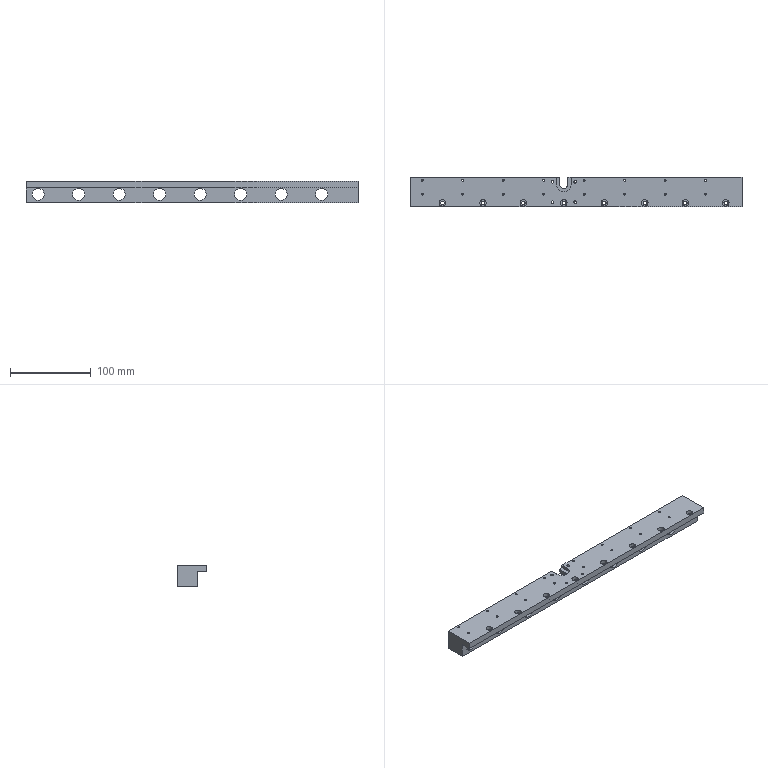Component | SolidWorks | 002MaterialPickingModuleA-1_004SidePlugModule-1_J-011-1 | 1 solid | 150 faces | box 410 x 37 x 26 mm | volume 255168 mm3 | cylinder 123 | plane 27 | commonest cylinder face diameters 2.5 x64 15 x16 8 x16 4.5 x16 3.3 x8 10 x1 18 x1 30 x1 | material 45
build123d program:
from build123d import *

# Parameters (mm, degrees)
SKETCH1_W                                       = 440
SKETCH1_H                                       = 37
BOSS_EXTRUDE1_DEPTH                             = 8
M4_HEX_SOCKET_HEAD_CAP_SCREW_CBORE1_D           = 4.5
M4_HEX_SOCKET_HEAD_CAP_SCREW_CBORE1_CBORE_D     = 8
M4_HEX_SOCKET_HEAD_CAP_SCREW_CBORE1_CBORE_DEPTH = 4.4
CUT_EXTRUDE1_DEPTH                              = 221.921
CUT_EXTRUDE2_DEPTH                              = 4
SKETCH7_W                                       = 440
SKETCH7_H                                       = 25
BOSS_EXTRUDE2_DEPTH                             = 18
CUT_EXTRUDE3_DEPTH                              = 16
HOLE1_D                                         = 15
HOLE1_DEPTH                                     = 93.98
CUT_EXTRUDE4_START                              = -10
CUT_EXTRUDE4_DEPTH                              = 10
M4_TAPPED_HOLE1_D                               = 3.3
SKETCH15_W                                      = 30
SKETCH15_H                                      = 37
CUT_EXTRUDE6_DEPTH                              = 223.302
M3_TAPPED_HOLE1_D                               = 2.5
LPATTERN1_COUNT                                 = 8
LPATTERN1_PITCH                                 = 50


with BuildPart() as part:
    # Sketch1 → Boss-Extrude1 (new body)
    with BuildSketch(Plane.XY):
        Rectangle(SKETCH1_W, SKETCH1_H)
    extrude(amount=BOSS_EXTRUDE1_DEPTH)

    # M4 Hex Socket Head Cap Screw CBORE1 (through all)
    with Locations(Plane.XY.offset(8)):
        with Locations((0, -13.5), (-50, -13.5), (-100, -13.5), (-150, -13.5), (50, -13.5), (100, -13.5), (150, -13.5), (-200, -13.5), (200, -13.5)):
            CounterBoreHole(M4_HEX_SOCKET_HEAD_CAP_SCREW_CBORE1_D / 2, M4_HEX_SOCKET_HEAD_CAP_SCREW_CBORE1_CBORE_D / 2, M4_HEX_SOCKET_HEAD_CAP_SCREW_CBORE1_CBORE_DEPTH)

    # Sketch5 → Cut-Extrude1 (cut, through all)
    with BuildSketch(Plane(origin=(0, 0, 0), x_dir=(-1, 0, 0), z_dir=(0, 0, -1))):
        with BuildLine():
            Line((5, 18.5), (5, 9.5))
            ThreePointArc((5, 9.5), (0, 4.5), (-5, 9.5))
            Line((-5, 9.5), (-5, 18.5))
            ThreePointArc((-5, 18.5), (0, 23.5), (5, 18.5))
        make_face()
    extrude(amount=-CUT_EXTRUDE1_DEPTH, mode=Mode.SUBTRACT)

    # Sketch6 → Cut-Extrude2 (cut)
    with BuildSketch(Plane.XY.offset(8)):
        with BuildLine():
            Line((-9, 9.5), (-9, 18.5))
            ThreePointArc((-9, 18.5), (0, 27.5), (9, 18.5))
            Line((9, 18.5), (9, 9.5))
            ThreePointArc((9, 9.5), (0, 0.5), (-9, 9.5))
        make_face()
    extrude(amount=-CUT_EXTRUDE2_DEPTH, mode=Mode.SUBTRACT)

    # Sketch7 → Boss-Extrude2 (add)
    with BuildSketch(Plane(origin=(0, 0, 0), x_dir=(-1, 0, 0), z_dir=(0, 0, -1))):
        with Locations((0, 6)):
            Rectangle(SKETCH7_W, SKETCH7_H)
    extrude(amount=BOSS_EXTRUDE2_DEPTH)

    # Sketch8 → Cut-Extrude3 (cut)
    with BuildSketch(Plane(origin=(0, 0, -18), x_dir=(-1, 0, 0), z_dir=(0, 0, -1))):
        with BuildLine():
            Line((-15, 9.5), (-15, 18.5))
            ThreePointArc((-15, 18.5), (0, 33.5), (15, 18.5))
            Line((15, 18.5), (15, 9.5))
            ThreePointArc((15, 9.5), (0, -5.5), (-15, 9.5))
        make_face()
    extrude(amount=-CUT_EXTRUDE3_DEPTH, mode=Mode.SUBTRACT)

    # Hole1
    with Locations(Plane(origin=(0, 18.5, 0), x_dir=(1, 0, 0), z_dir=(0, 1, 0))):
        with Locations((25, 8), (-25, 8), (-75, 8), (75, 8), (-125, 8), (-175, 8), (125, 8), (175, 8)):
            Hole(HOLE1_D / 2, depth=HOLE1_DEPTH)

    # Sketch11 → Cut-Extrude4 (cut)
    with BuildSketch(Plane.XY.offset(CUT_EXTRUDE4_START)):
        with BuildLine():
            Line((-5, 18.5), (5, 18.5))
            Line((5, 18.5), (5, 9.5))
            ThreePointArc((5, 9.5), (0, 4.5), (-5, 9.5))
            Line((-5, 9.5), (-5, 18.5))
        make_face()
    extrude(amount=CUT_EXTRUDE4_DEPTH, mode=Mode.SUBTRACT)

    # M4 Tapped Hole1 (through all)
    with Locations(Plane.XY.offset(8)):
        with Locations((-14, 12.5), (14, 12.5), (-14, -12.5), (14, -12.5)):
            Hole(M4_TAPPED_HOLE1_D / 2)

    # Sketch15 → Cut-Extrude6 (cut, through all)
    with BuildSketch(Plane.XY.offset(8)):
        with Locations((-205, 0)):
            Rectangle(SKETCH15_W, SKETCH15_H)
    extrude(amount=-CUT_EXTRUDE6_DEPTH, mode=Mode.SUBTRACT)

    # M3 Tapped Hole1 (through all)
    with Locations(Plane.XY.offset(8)):
        with Locations((-175, 14.5), (-175, -2.5)):
            m3_tapped_hole1 = Hole(M3_TAPPED_HOLE1_D / 2)

    # LPattern1: M3 Tapped Hole1 ×8
    with Locations(*[(i * LPATTERN1_PITCH, 0, 0) for i in range(1, LPATTERN1_COUNT)]):
        add(m3_tapped_hole1, mode=Mode.SUBTRACT)


solid = part.part

# Placed as in the assembly
solid = solid.moved(Location((220.324, 309.519, 472.731), (0, 0, 0)))